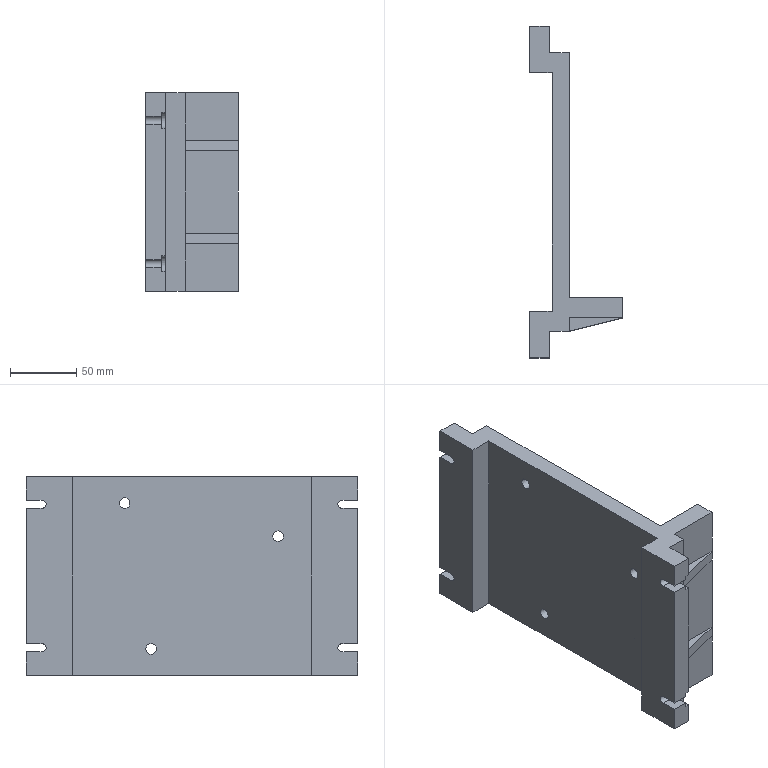Component | NX | JIG_BODY | 1 solid | 77 faces | volume 654693 mm3 | plane 52 | cylinder 18 | cone 7 | commonest cylinder face diameters 8 x10 12 x4 6 x4